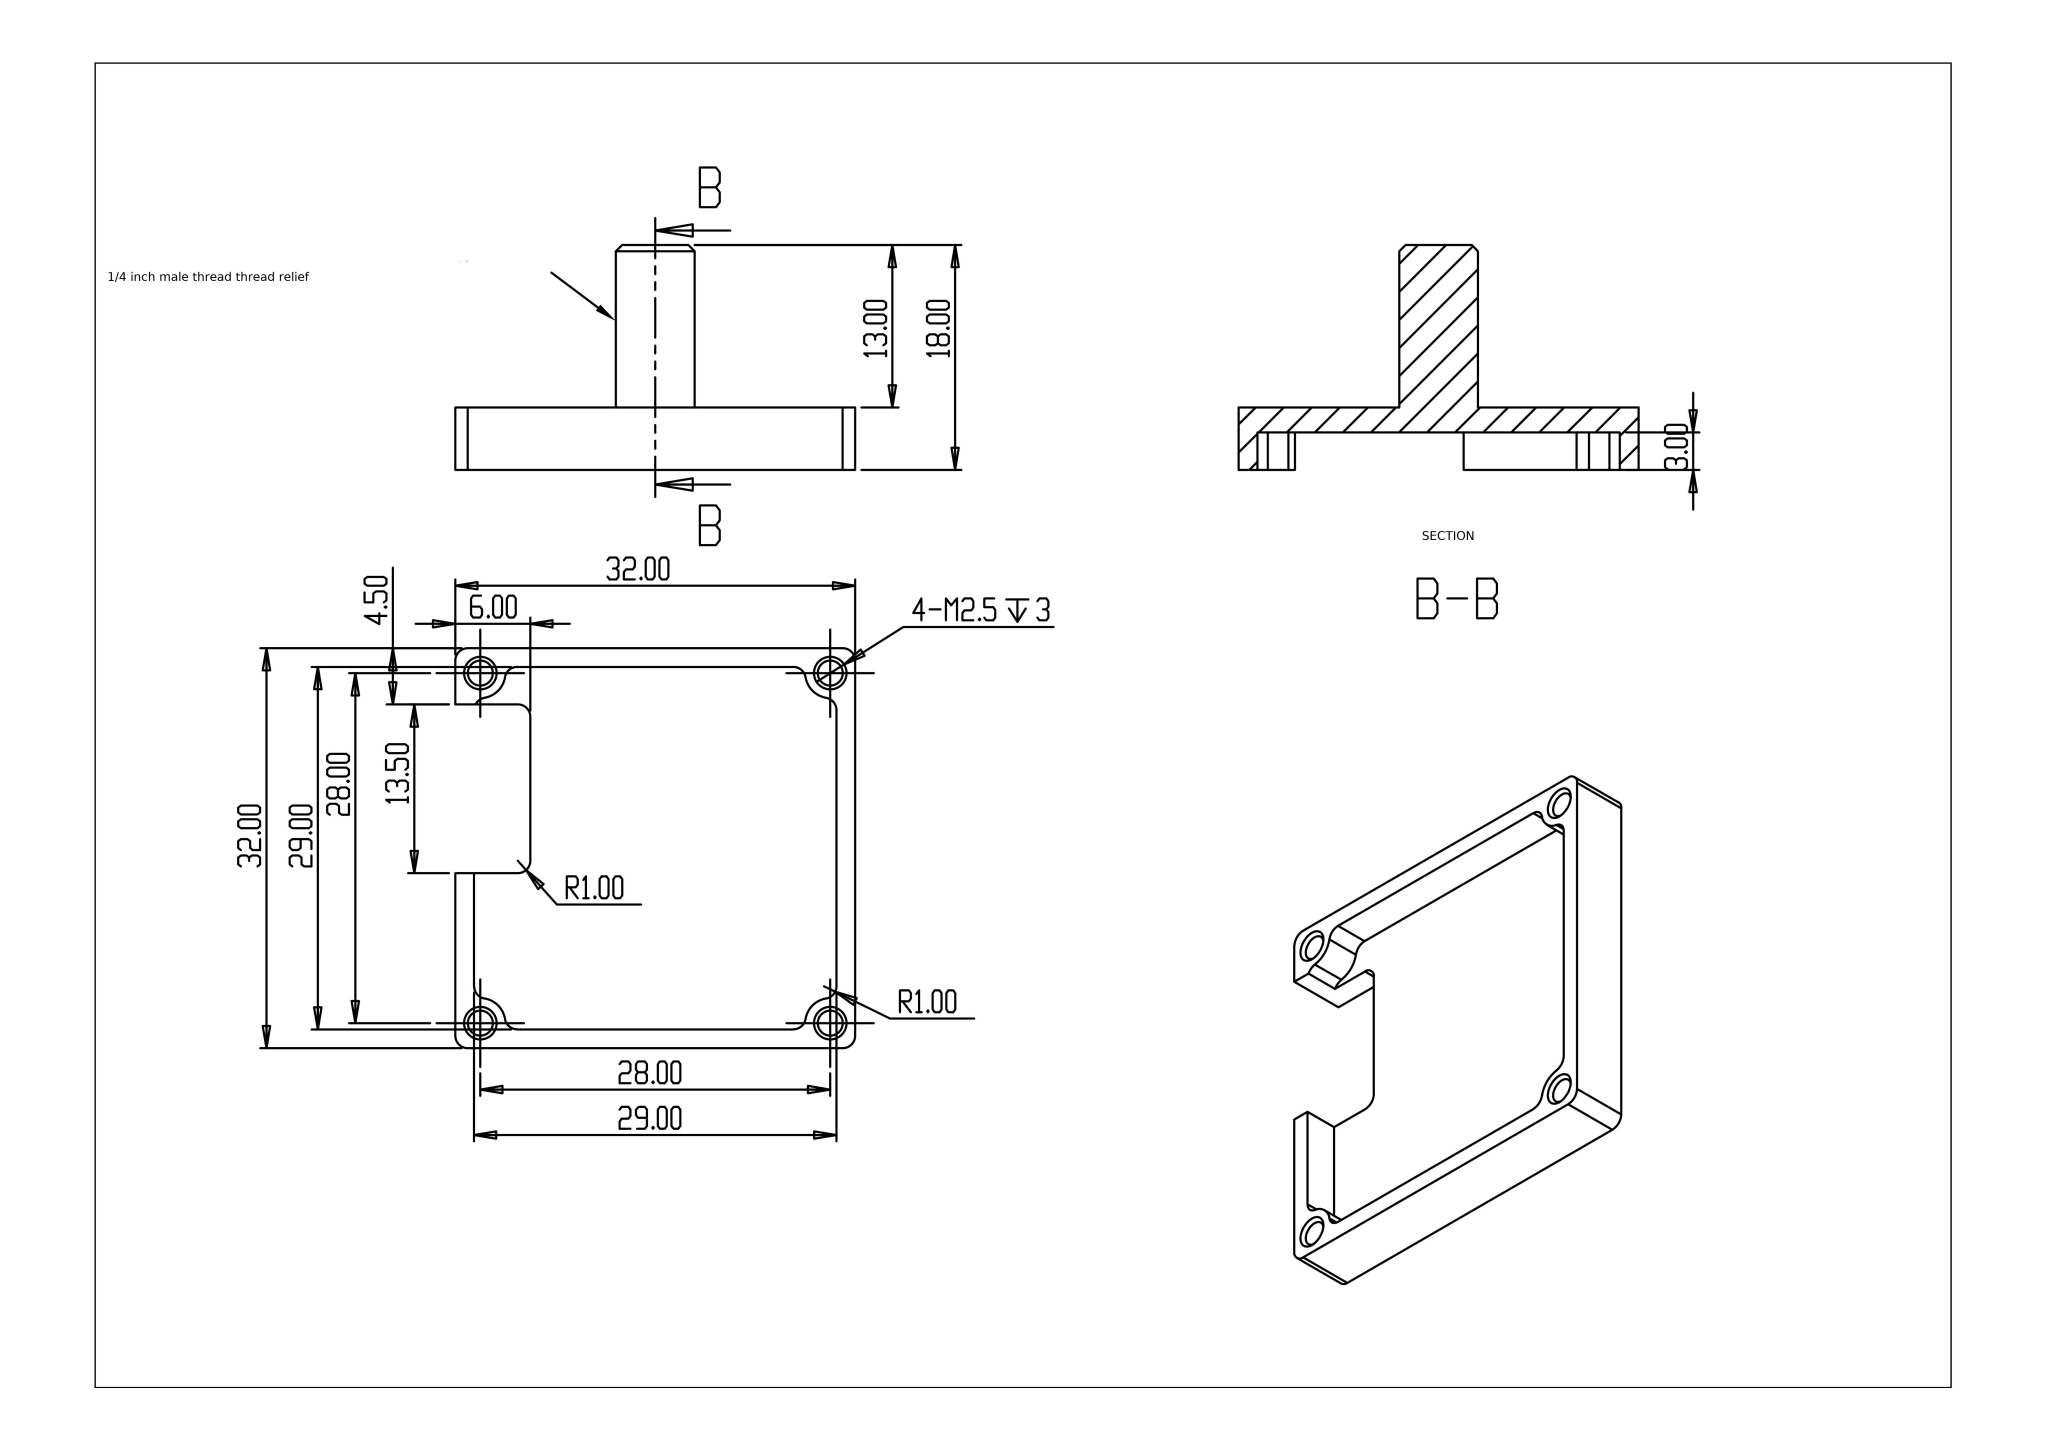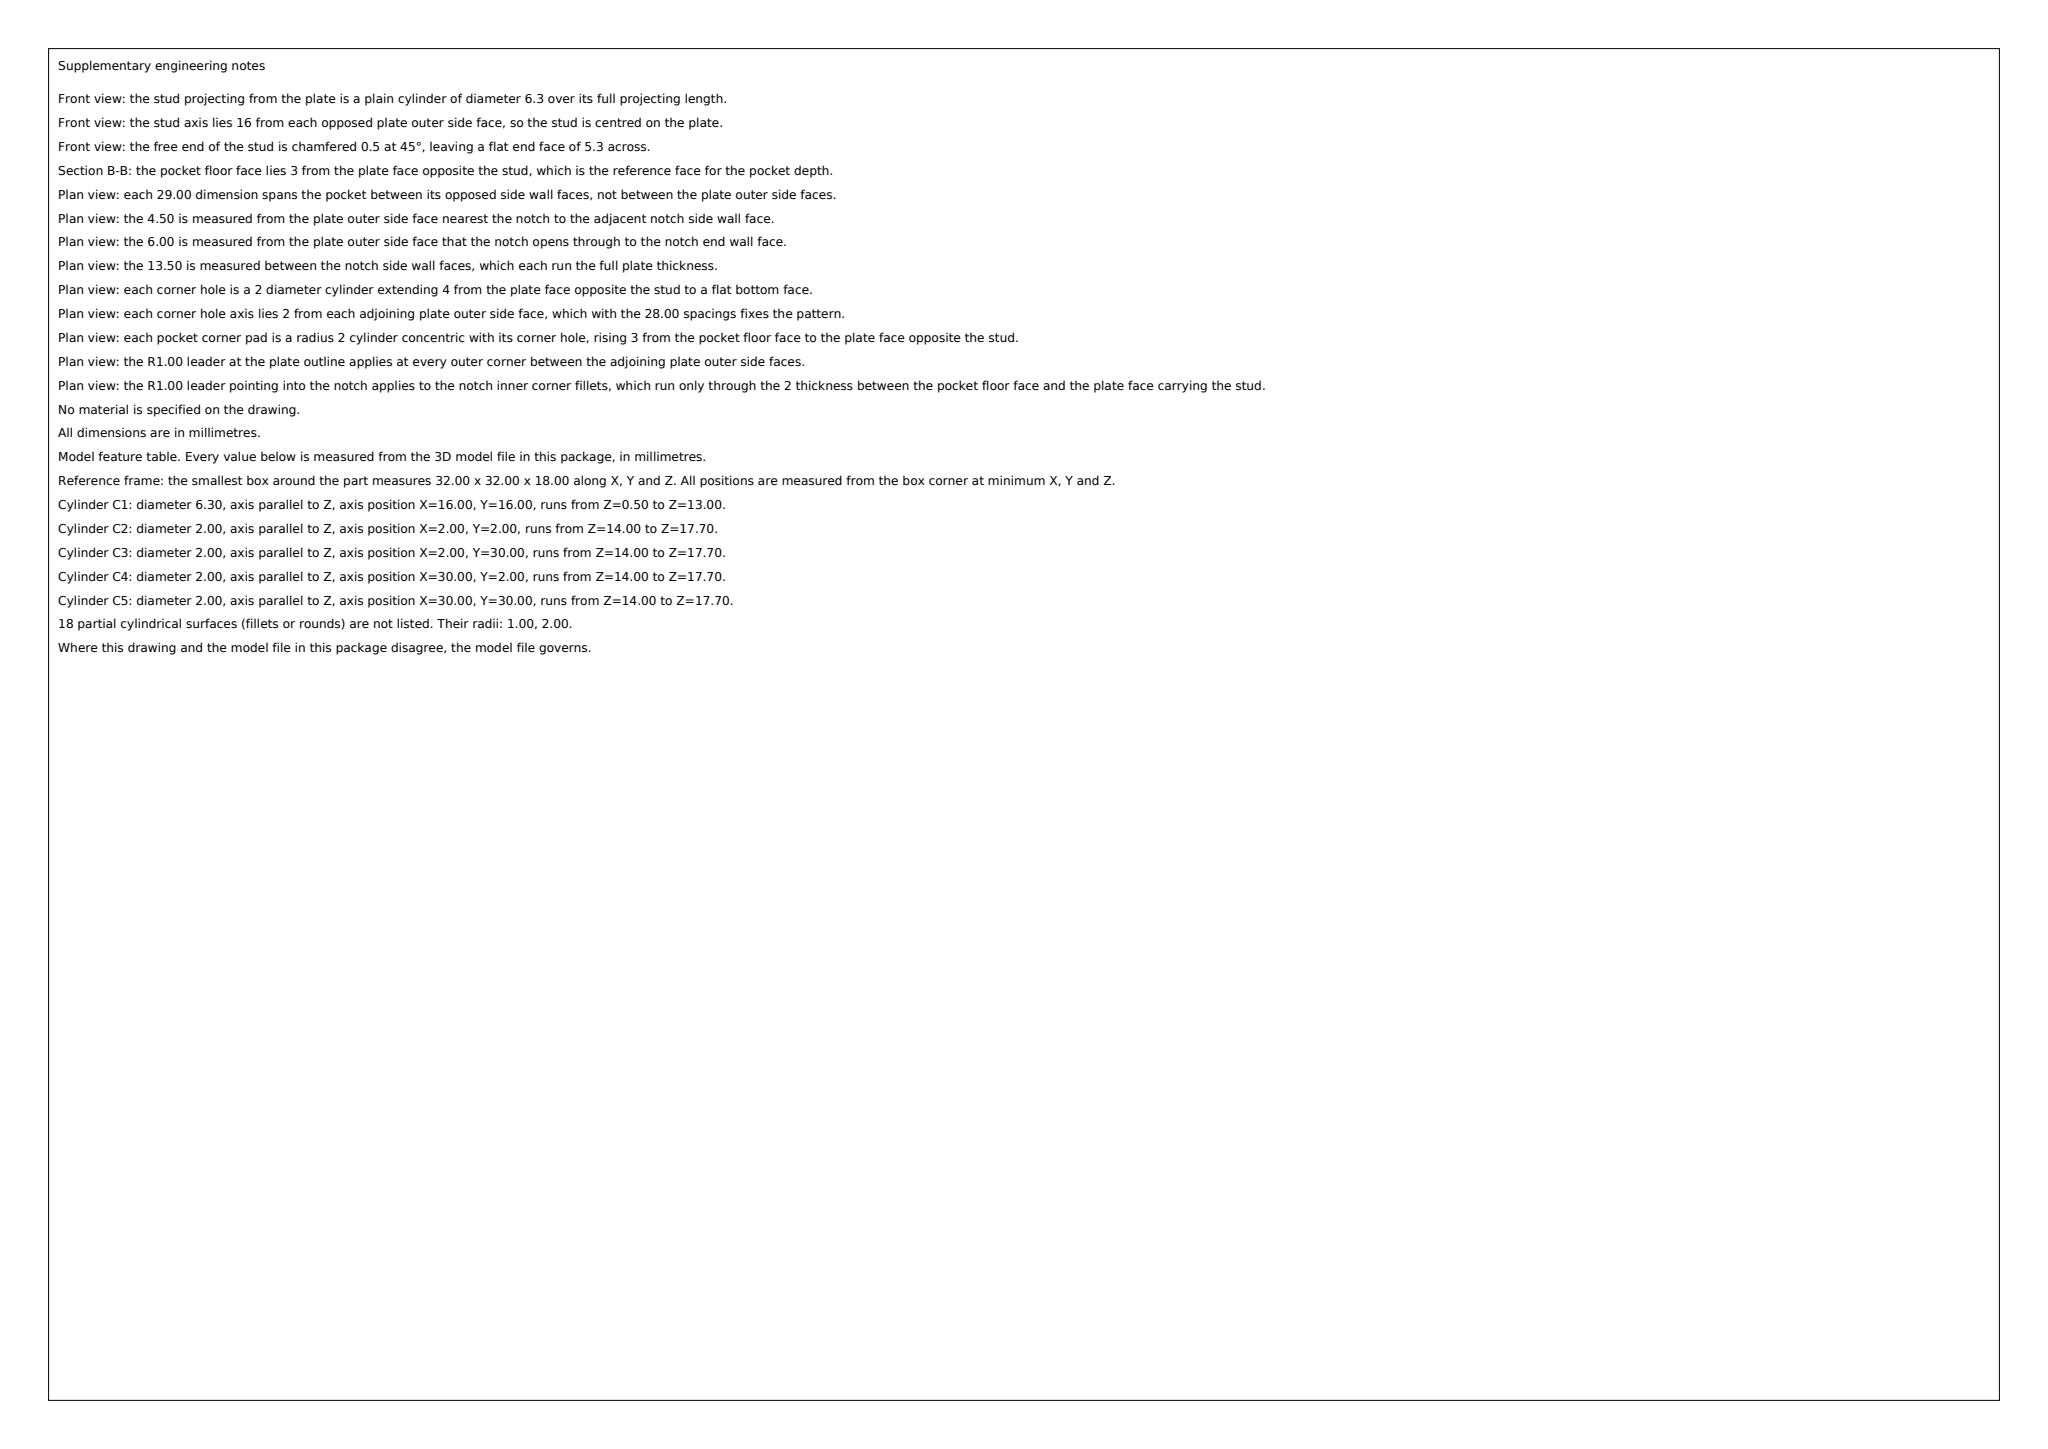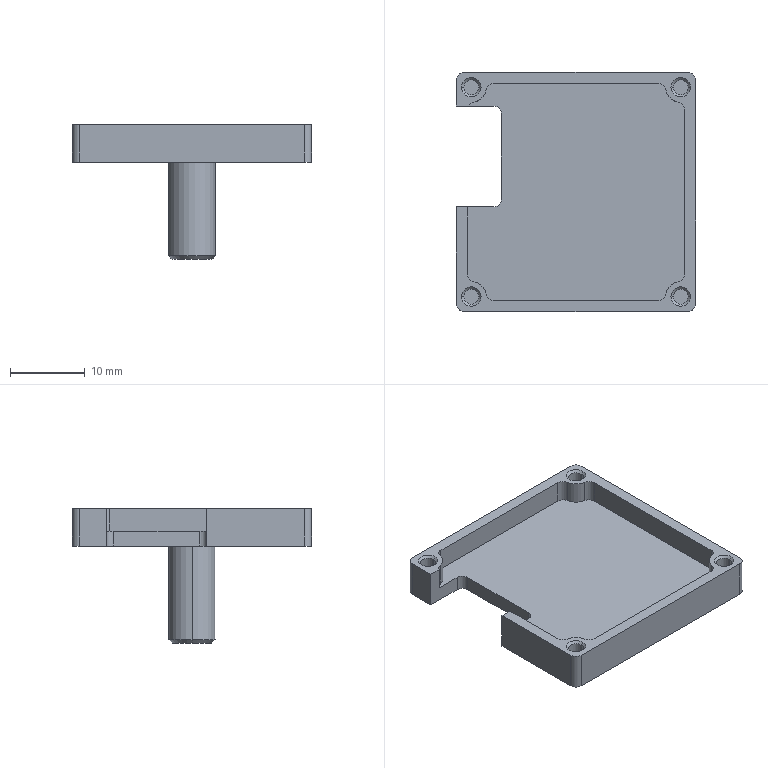Part | SolidWorks | mm | 1 solid | 58 faces | box 32 x 32 x 18 mm | volume 2791 mm3 | cylinder 28 | plane 20 | cone 10 | commonest cylinder face diameters 2 x22 4 x4 6.3 x2
Drawing notes:
STUD END CHAMFER: Ø6.3 TO Ø5.3, 90° INCL (0.5 X 45°) | from the solid: cones [90.0, ref_dia 5.3] on Ø6.3 stud (cyl dia 6.3, axis z, pos 16,16)
THD RELIEF AT STUD BASE: Ø5.3 X 0.5 WIDE, 90° INCL CONE | from the solid: 2nd 90° cone at ref_dia 5.3 on Ø6.3 x 12.5 stud; 13.0 stud length minus 12.5 cyl
LOWER RECESS FLOOR 4.00 DEEP FROM TOP FACE (1.00 STEP) | from the solid: z planes at 18.0 (top), 15.0 (3.00 pocket floor), 14.0 (lower floor)
STUD Ø6.3 AXIS CTRD ON PLATE: 16.00 FROM EACH 32.00 EDGE | from the solid: cyl dia 6.3 axis z at (16.0,16.0); bbox 32x32x18
1/4 MALE THD ON Ø6.3 STUD, THD LG 12.5, C0.5 AT FREE END | from the solid: cyl [6.3,z,(16,16),12.5]; cone 90 deg ref dia 5.3 at stud end
4X Ø4.00 CORNER BOSS/PAD AT M2.5 HOLES, AXES 2.00 FROM EACH ADJACENT 32.00 EDGE; 3.00 AXIAL LENGTH, TOP FLUSH WITH PLATE TOP FACE (EXTENDS 3.00 DOWN TO THE 3.00 STEP FLOOR) | from the solid: cylinders dia 4.0 axis z at (2,2),(2,30),(30,2),(30,30) length 3.0; z planes at 15.0 and 18.0
4X R1.00 EXTERNAL CORNER ROUND ON 32.00 X 32.00 PLATE, CENTERS 1.00 FROM EACH 32.00 EDGE, FULL 5.00 PLATE THICKNESS | from the solid: cylinders dia 2.0 axis z at (1,1),(1,31),(31,1),(31,31) length 5.0; z planes 13.0 and 18.0
build123d program:
from build123d import *

# Parameters (mm, degrees)
BOSS_EXTRUDE1_DEPTH = 5
CUT_EXTRUDE1_START  = -3
CUT_EXTRUDE1_DEPTH  = 3
CUT_EXTRUDE2_DEPTH  = 4
CHAMFER1_SIZE       = 0.3
SKETCH5_R           = 3.15
BOSS_EXTRUDE2_DEPTH = 13
CHAMFER2_SIZE       = 0.5


with BuildPart() as part:
    # Sketch1 → Boss-Extrude1 (new body)
    with BuildSketch(Plane.XY):
        with BuildLine():
            Line((-14.389, 11.5), (-11, 11.5))
            ThreePointArc((-11, 11.5), (-10.293, 11.207), (-10, 10.5))
            Line((-10, 10.5), (-10, -1))
            ThreePointArc((-10, -1), (-10.293, -1.707), (-11, -2))
            Line((-11, -2), (-14.5, -2))
            Line((-14.5, -2), (-16, -2))
            Line((-16, -2), (-16, -15))
            ThreePointArc((-16, -15), (-15.707, -15.707), (-15, -16))
            Line((-15, -16), (15, -16))
            ThreePointArc((15, -16), (15.707, -15.707), (16, -15))
            Line((16, -15), (16, 15))
            ThreePointArc((16, 15), (15.707, 15.707), (15, 16))
            Line((15, 16), (-15, 16))
            ThreePointArc((-15, 16), (-15.707, 15.707), (-16, 15))
            Line((-16, 15), (-16, 11.5))
            Line((-16, 11.5), (-14.389, 11.5))
        make_face()
    extrude(amount=BOSS_EXTRUDE1_DEPTH)

    # Sketch2 → Cut-Extrude1 (cut)
    with BuildSketch(Plane.XY.offset(5).offset(CUT_EXTRUDE1_START)):
        with BuildLine():
            ThreePointArc((-13.667, 12.028), (-14.09, 11.849), (-14.389, 11.5))
            Line((-14.389, 11.5), (-11, 11.5))
            ThreePointArc((-11, 11.5), (-10.293, 11.207), (-10, 10.5))
            Line((-10, 10.5), (-10, -1))
            ThreePointArc((-10, -1), (-10.293, -1.707), (-11, -2))
            Line((-11, -2), (-14.5, -2))
            Line((-14.5, -2), (-14.5, -11.042))
            ThreePointArc((-14.5, -11.042), (-14.264, -11.687), (-13.667, -12.028))
            ThreePointArc((-13.667, -12.028), (-12.586, -12.586), (-12.028, -13.667))
            ThreePointArc((-12.028, -13.667), (-11.687, -14.264), (-11.042, -14.5))
            Line((-11.042, -14.5), (11.042, -14.5))
            ThreePointArc((11.042, -14.5), (11.687, -14.264), (12.028, -13.667))
            ThreePointArc((12.028, -13.667), (12.586, -12.586), (13.667, -12.028))
            ThreePointArc((13.667, -12.028), (14.264, -11.687), (14.5, -11.042))
            Line((14.5, -11.042), (14.5, 11.042))
            ThreePointArc((14.5, 11.042), (14.264, 11.687), (13.667, 12.028))
            ThreePointArc((13.667, 12.028), (12.586, 12.586), (12.028, 13.667))
            ThreePointArc((12.028, 13.667), (11.687, 14.264), (11.042, 14.5))
            Line((11.042, 14.5), (-11.042, 14.5))
            ThreePointArc((-11.042, 14.5), (-11.687, 14.264), (-12.028, 13.667))
            ThreePointArc((-12.028, 13.667), (-12.586, 12.586), (-13.667, 12.028))
        make_face()
    extrude(amount=CUT_EXTRUDE1_DEPTH, mode=Mode.SUBTRACT)

    # Sketch4 → Cut-Extrude2 (cut)
    with BuildSketch(Plane.XY.offset(5)):
        with BuildLine():
            ThreePointArc((-14, 15), (-15, 14), (-14, 13))
            ThreePointArc((-14, 13), (-13, 14), (-14, 15))
        make_face()
        with BuildLine():
            ThreePointArc((14, 15), (13, 14), (14, 13))
            ThreePointArc((14, 13), (15, 14), (14, 15))
        make_face()
        with BuildLine():
            ThreePointArc((14, -13), (13, -14), (14, -15))
            ThreePointArc((14, -15), (15, -14), (14, -13))
        make_face()
        with BuildLine():
            ThreePointArc((-14, -13), (-15, -14), (-14, -15))
            ThreePointArc((-14, -15), (-13, -14), (-14, -13))
        make_face()
    extrude(amount=-CUT_EXTRUDE2_DEPTH, mode=Mode.SUBTRACT)

    # Chamfer1
    chamfer1_edges = [part.edges().sort_by_distance(p)[0] for p in [
        (-14, -15, 5),
        (14, -15, 5),
        (14, 15, 5),
        (-14, 13, 5),
    ]]
    chamfer(chamfer1_edges, length=CHAMFER1_SIZE)

    # Sketch5 → Boss-Extrude2 (add)
    with BuildSketch(Plane(origin=(0, 0, 0), x_dir=(-1, 0, 0), z_dir=(0, 0, -1))):
        with Locations(Location((0, 0, 0), (0, 0, 180))):
            Circle(SKETCH5_R)
    extrude(amount=BOSS_EXTRUDE2_DEPTH)

    # Chamfer2
    chamfer2_edges = [part.edges().sort_by_distance(p)[0] for p in [
        (-3.15, 0, -13),
    ]]
    chamfer(chamfer2_edges, length=CHAMFER2_SIZE)


solid = part.part